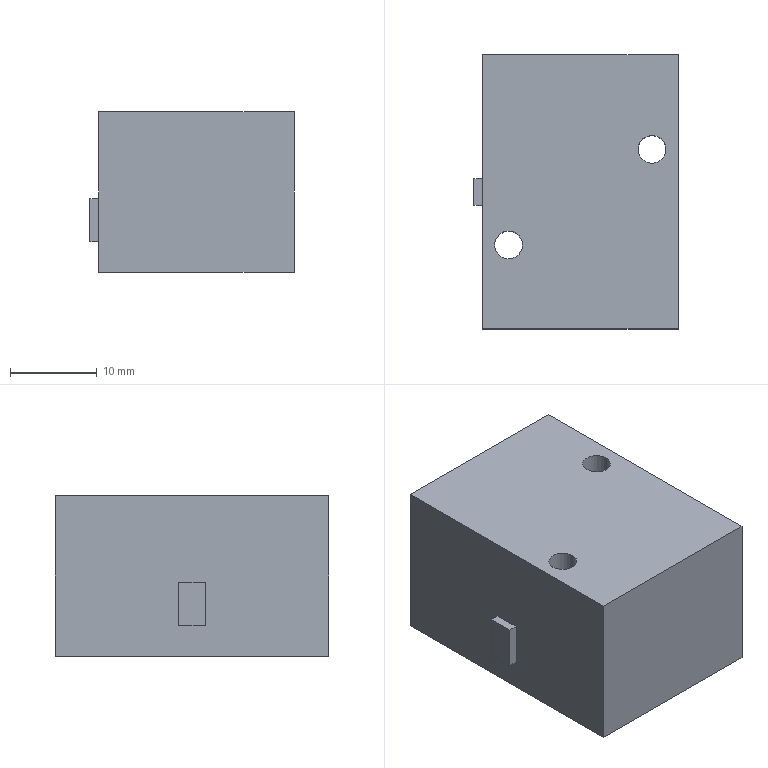Component | SolidWorks | CLS-MechanismAuxiliarySwitch-1 | 1 solid | 15 faces | box 23.5 x 31.5 x 18.5 mm | volume 12829 mm3 | plane 11 | cylinder 4 | commonest cylinder face diameters 3.2 x4 | material 2.0 Galvanized Sheet Q235A
build123d program:
from build123d import *

# Parameters (mm, degrees)
SKETCH1_W            = 22.5
SKETCH1_H            = 31.5
BOSS_EXTRUDE1_DEPTH  = 18.5
SKETCH2_R            = 1.6
CUT_EXTRUDE1_DEPTH   = 27.775
LPATTERN1_COUNT      = 2
LPATTERN1_PITCH      = 16.5
LPATTERN1_COUNT_DIR2 = 2
LPATTERN1_PITCH_DIR2 = 11
SKETCH3_W            = 5
SKETCH3_H            = 3
BOSS_EXTRUDE2_DEPTH  = 1


with BuildPart() as part:
    # Sketch1 → Boss-Extrude1 (new body)
    with BuildSketch(Plane.XY):
        Rectangle(SKETCH1_W, SKETCH1_H)
    extrude(amount=BOSS_EXTRUDE1_DEPTH)

    # Sketch2 → Cut-Extrude1 (cut, through all)
    with BuildSketch(Plane(origin=(0, 0, 0), x_dir=(-1, 0, 0), z_dir=(0, 0, -1))):
        with Locations((-8.25, 4.891)):
            Circle(SKETCH2_R)
    cut_extrude1 = extrude(amount=-CUT_EXTRUDE1_DEPTH, mode=Mode.SUBTRACT)

    # LPattern1: Cut-Extrude1 2 × 2, 2 skipped
    with Locations(*[(-i * LPATTERN1_PITCH, -j * LPATTERN1_PITCH_DIR2, 0) for i in range(LPATTERN1_COUNT) for j in range(LPATTERN1_COUNT_DIR2) if (i, j) not in ((0, 0), (0, 1), (1, 0))]):
        add(cut_extrude1, mode=Mode.SUBTRACT)

    # Sketch3 → Boss-Extrude2 (add)
    with BuildSketch(Plane.ZY.offset(11.25)):
        with Locations((6, 0)):
            Rectangle(SKETCH3_W, SKETCH3_H)
    extrude(amount=BOSS_EXTRUDE2_DEPTH)


solid = part.part

# Placed as in the assembly
solid = solid.moved(Location((19.224, 11.301, -21.501), (0, 0, 0)))
STEP:
#1=COLOUR_RGB('',0.7922,0.8196,0.9333);
#2=FILL_AREA_STYLE_COLOUR('',#1);
#3=FILL_AREA_STYLE('',(#2));
#4=SURFACE_STYLE_FILL_AREA(#3);
#5=SURFACE_SIDE_STYLE('',(#4));
#6=SURFACE_STYLE_USAGE(.BOTH.,#5);
#7=PRESENTATION_STYLE_ASSIGNMENT((#6));
#8=CARTESIAN_POINT('',(0.495,0.2044,-0.1181));
#9=VERTEX_POINT('',#8);
#10=CARTESIAN_POINT('',(0.369,0.2044,-0.1181));
#11=VERTEX_POINT('',#10);
#12=CARTESIAN_POINT('',(0.432,0.2044,-0.1181));
#13=DIRECTION('',(0.,0.,-1.));
#14=DIRECTION('',(-1.,0.,0.));
#15=AXIS2_PLACEMENT_3D('',#12,#13,#14);
#16=CIRCLE('',#15,0.06299);
#17=EDGE_CURVE('',#9,#11,#16,.T.);
#18=ORIENTED_EDGE('',*,*,#17,.F.);
#19=CARTESIAN_POINT('',(0.495,0.2044,-0.8465));
#20=VERTEX_POINT('',#19);
#21=CARTESIAN_POINT('',(0.495,0.2044,-0.1181));
#22=DIRECTION('',(0.,0.,-1.));
#23=VECTOR('',#22,39.37);
#24=LINE('',#21,#23);
#25=EDGE_CURVE('',#9,#20,#24,.T.);
#26=ORIENTED_EDGE('',*,*,#25,.T.);
#27=CARTESIAN_POINT('',(0.369,0.2044,-0.8465));
#28=VERTEX_POINT('',#27);
#29=CARTESIAN_POINT('',(0.432,0.2044,-0.8465));
#30=DIRECTION('',(0.,0.,-1.));
#31=DIRECTION('',(-1.,0.,0.));
#32=AXIS2_PLACEMENT_3D('',#29,#30,#31);
#33=CIRCLE('',#32,0.06299);
#34=EDGE_CURVE('',#20,#28,#33,.T.);
#35=ORIENTED_EDGE('',*,*,#34,.T.);
#36=CARTESIAN_POINT('',(0.369,0.2044,-0.1181));
#37=DIRECTION('',(0.,0.,-1.));
#38=VECTOR('',#37,39.37);
#39=LINE('',#36,#38);
#40=EDGE_CURVE('',#11,#28,#39,.T.);
#41=ORIENTED_EDGE('',*,*,#40,.F.);
#42=EDGE_LOOP('',(#18,#26,#35,#41));
#43=FACE_OUTER_BOUND('',#42,.T.);
#44=CARTESIAN_POINT('',(0.432,0.2044,-0.1181));
#45=DIRECTION('',(0.,0.,-1.));
#46=DIRECTION('',(-1.,0.,0.));
#47=AXIS2_PLACEMENT_3D('',#44,#45,#46);
#48=CYLINDRICAL_SURFACE('',#47,0.06299);
#49=ADVANCED_FACE('',(#43),#48,.F.);
#50=CARTESIAN_POINT('',(1.145,0.6375,-0.1181));
#51=VERTEX_POINT('',#50);
#52=CARTESIAN_POINT('',(1.019,0.6375,-0.1181));
#53=VERTEX_POINT('',#52);
#54=CARTESIAN_POINT('',(1.082,0.6375,-0.1181));
#55=DIRECTION('',(0.,0.,-1.));
#56=DIRECTION('',(-1.,0.,0.));
#57=AXIS2_PLACEMENT_3D('',#54,#55,#56);
#58=CIRCLE('',#57,0.06299);
#59=EDGE_CURVE('',#51,#53,#58,.T.);
#60=ORIENTED_EDGE('',*,*,#59,.F.);
#61=CARTESIAN_POINT('',(1.145,0.6375,-0.8465));
#62=VERTEX_POINT('',#61);
#63=CARTESIAN_POINT('',(1.145,0.6375,-0.1181));
#64=DIRECTION('',(0.,0.,-1.));
#65=VECTOR('',#64,39.37);
#66=LINE('',#63,#65);
#67=EDGE_CURVE('',#51,#62,#66,.T.);
#68=ORIENTED_EDGE('',*,*,#67,.T.);
#69=CARTESIAN_POINT('',(1.019,0.6375,-0.8465));
#70=VERTEX_POINT('',#69);
#71=CARTESIAN_POINT('',(1.082,0.6375,-0.8465));
#72=DIRECTION('',(0.,0.,-1.));
#73=DIRECTION('',(-1.,0.,0.));
#74=AXIS2_PLACEMENT_3D('',#71,#72,#73);
#75=CIRCLE('',#74,0.06299);
#76=EDGE_CURVE('',#62,#70,#75,.T.);
#77=ORIENTED_EDGE('',*,*,#76,.T.);
#78=CARTESIAN_POINT('',(1.019,0.6375,-0.1181));
#79=DIRECTION('',(0.,0.,-1.));
#80=VECTOR('',#79,39.37);
#81=LINE('',#78,#80);
#82=EDGE_CURVE('',#53,#70,#81,.T.);
#83=ORIENTED_EDGE('',*,*,#82,.F.);
#84=EDGE_LOOP('',(#60,#68,#77,#83));
#85=FACE_OUTER_BOUND('',#84,.T.);
#86=CARTESIAN_POINT('',(1.082,0.6375,-0.1181));
#87=DIRECTION('',(0.,0.,-1.));
#88=DIRECTION('',(-1.,0.,0.));
#89=AXIS2_PLACEMENT_3D('',#86,#87,#88);
#90=CYLINDRICAL_SURFACE('',#89,0.06299);
#91=ADVANCED_FACE('',(#85),#90,.F.);
#92=CARTESIAN_POINT('',(0.3139,1.065,-0.8465));
#93=VERTEX_POINT('',#92);
#94=CARTESIAN_POINT('',(0.3139,-0.1752,-0.8465));
#95=VERTEX_POINT('',#94);
#96=CARTESIAN_POINT('',(0.3139,1.065,-0.8465));
#97=DIRECTION('',(0.,-1.,0.));
#98=VECTOR('',#97,39.37);
#99=LINE('',#96,#98);
#100=EDGE_CURVE('',#93,#95,#99,.T.);
#101=ORIENTED_EDGE('',*,*,#100,.T.);
#102=CARTESIAN_POINT('',(0.3139,-0.1752,-0.1181));
#103=VERTEX_POINT('',#102);
#104=CARTESIAN_POINT('',(0.3139,-0.1752,-0.1181));
#105=DIRECTION('',(0.,0.,-1.));
#106=VECTOR('',#105,39.37);
#107=LINE('',#104,#106);
#108=EDGE_CURVE('',#103,#95,#107,.T.);
#109=ORIENTED_EDGE('',*,*,#108,.F.);
#110=CARTESIAN_POINT('',(0.3139,1.065,-0.1181));
#111=VERTEX_POINT('',#110);
#112=CARTESIAN_POINT('',(0.3139,1.065,-0.1181));
#113=DIRECTION('',(0.,-1.,0.));
#114=VECTOR('',#113,39.37);
#115=LINE('',#112,#114);
#116=EDGE_CURVE('',#111,#103,#115,.T.);
#117=ORIENTED_EDGE('',*,*,#116,.F.);
#118=CARTESIAN_POINT('',(0.3139,1.065,-0.1181));
#119=DIRECTION('',(0.,0.,-1.));
#120=VECTOR('',#119,39.37);
#121=LINE('',#118,#120);
#122=EDGE_CURVE('',#111,#93,#121,.T.);
#123=ORIENTED_EDGE('',*,*,#122,.T.);
#124=EDGE_LOOP('',(#101,#109,#117,#123));
#125=FACE_OUTER_BOUND('',#124,.T.);
#126=CARTESIAN_POINT('',(0.3139,0.3859,-0.5118));
#127=VERTEX_POINT('',#126);
#128=CARTESIAN_POINT('',(0.3139,0.504,-0.5118));
#129=VERTEX_POINT('',#128);
#130=CARTESIAN_POINT('',(0.3139,0.504,-0.5118));
#131=DIRECTION('',(0.,1.,-0.));
#132=VECTOR('',#131,39.37);
#133=LINE('',#130,#132);
#134=EDGE_CURVE('',#127,#129,#133,.T.);
#135=ORIENTED_EDGE('',*,*,#134,.F.);
#136=CARTESIAN_POINT('',(0.3139,0.3859,-0.7087));
#137=VERTEX_POINT('',#136);
#138=CARTESIAN_POINT('',(0.3139,0.3859,-0.7087));
#139=DIRECTION('',(0.,0.,1.));
#140=VECTOR('',#139,39.37);
#141=LINE('',#138,#140);
#142=EDGE_CURVE('',#137,#127,#141,.T.);
#143=ORIENTED_EDGE('',*,*,#142,.F.);
#144=CARTESIAN_POINT('',(0.3139,0.504,-0.7087));
#145=VERTEX_POINT('',#144);
#146=CARTESIAN_POINT('',(0.3139,0.504,-0.7087));
#147=DIRECTION('',(0.,-1.,0.));
#148=VECTOR('',#147,39.37);
#149=LINE('',#146,#148);
#150=EDGE_CURVE('',#145,#137,#149,.T.);
#151=ORIENTED_EDGE('',*,*,#150,.F.);
#152=CARTESIAN_POINT('',(0.3139,0.504,-0.7087));
#153=DIRECTION('',(0.,0.,-1.));
#154=VECTOR('',#153,39.37);
#155=LINE('',#152,#154);
#156=EDGE_CURVE('',#129,#145,#155,.T.);
#157=ORIENTED_EDGE('',*,*,#156,.F.);
#158=EDGE_LOOP('',(#135,#143,#151,#157));
#159=FACE_BOUND('',#158,.T.);
#160=CARTESIAN_POINT('',(0.3139,1.065,-0.1181));
#161=DIRECTION('',(1.,0.,0.));
#162=DIRECTION('',(-0.,1.,0.));
#163=AXIS2_PLACEMENT_3D('',#160,#161,#162);
#164=PLANE('',#163);
#165=ADVANCED_FACE('',(#125,#159),#164,.F.);
#166=CARTESIAN_POINT('',(1.2,-0.1752,-0.8465));
#167=VERTEX_POINT('',#166);
#168=CARTESIAN_POINT('',(1.2,-0.1752,-0.8465));
#169=DIRECTION('',(1.,0.,0.));
#170=VECTOR('',#169,39.37);
#171=LINE('',#168,#170);
#172=EDGE_CURVE('',#95,#167,#171,.T.);
#173=ORIENTED_EDGE('',*,*,#172,.T.);
#174=CARTESIAN_POINT('',(1.2,-0.1752,-0.1181));
#175=VERTEX_POINT('',#174);
#176=CARTESIAN_POINT('',(1.2,-0.1752,-0.1181));
#177=DIRECTION('',(0.,0.,-1.));
#178=VECTOR('',#177,39.37);
#179=LINE('',#176,#178);
#180=EDGE_CURVE('',#175,#167,#179,.T.);
#181=ORIENTED_EDGE('',*,*,#180,.F.);
#182=CARTESIAN_POINT('',(1.2,-0.1752,-0.1181));
#183=DIRECTION('',(1.,0.,0.));
#184=VECTOR('',#183,39.37);
#185=LINE('',#182,#184);
#186=EDGE_CURVE('',#103,#175,#185,.T.);
#187=ORIENTED_EDGE('',*,*,#186,.F.);
#188=ORIENTED_EDGE('',*,*,#108,.T.);
#189=EDGE_LOOP('',(#173,#181,#187,#188));
#190=FACE_OUTER_BOUND('',#189,.T.);
#191=CARTESIAN_POINT('',(1.2,-0.1752,-0.1181));
#192=DIRECTION('',(0.,1.,0.));
#193=DIRECTION('',(0.,0.,1.));
#194=AXIS2_PLACEMENT_3D('',#191,#192,#193);
#195=PLANE('',#194);
#196=ADVANCED_FACE('',(#190),#195,.F.);
#197=CARTESIAN_POINT('',(1.2,1.065,-0.8465));
#198=VERTEX_POINT('',#197);
#199=CARTESIAN_POINT('',(1.2,1.065,-0.8465));
#200=DIRECTION('',(-0.,1.,0.));
#201=VECTOR('',#200,39.37);
#202=LINE('',#199,#201);
#203=EDGE_CURVE('',#167,#198,#202,.T.);
#204=ORIENTED_EDGE('',*,*,#203,.T.);
#205=CARTESIAN_POINT('',(1.2,1.065,-0.1181));
#206=VERTEX_POINT('',#205);
#207=CARTESIAN_POINT('',(1.2,1.065,-0.1181));
#208=DIRECTION('',(0.,0.,-1.));
#209=VECTOR('',#208,39.37);
#210=LINE('',#207,#209);
#211=EDGE_CURVE('',#206,#198,#210,.T.);
#212=ORIENTED_EDGE('',*,*,#211,.F.);
#213=CARTESIAN_POINT('',(1.2,1.065,-0.1181));
#214=DIRECTION('',(-0.,1.,0.));
#215=VECTOR('',#214,39.37);
#216=LINE('',#213,#215);
#217=EDGE_CURVE('',#175,#206,#216,.T.);
#218=ORIENTED_EDGE('',*,*,#217,.F.);
#219=ORIENTED_EDGE('',*,*,#180,.T.);
#220=EDGE_LOOP('',(#204,#212,#218,#219));
#221=FACE_OUTER_BOUND('',#220,.T.);
#222=CARTESIAN_POINT('',(1.2,1.065,-0.1181));
#223=DIRECTION('',(-1.,-0.,0.));
#224=DIRECTION('',(0.,-1.,0.));
#225=AXIS2_PLACEMENT_3D('',#222,#223,#224);
#226=PLANE('',#225);
#227=ADVANCED_FACE('',(#221),#226,.F.);
#228=CARTESIAN_POINT('',(1.2,1.065,-0.8465));
#229=DIRECTION('',(-1.,-0.,0.));
#230=VECTOR('',#229,39.37);
#231=LINE('',#228,#230);
#232=EDGE_CURVE('',#198,#93,#231,.T.);
#233=ORIENTED_EDGE('',*,*,#232,.T.);
#234=ORIENTED_EDGE('',*,*,#122,.F.);
#235=CARTESIAN_POINT('',(1.2,1.065,-0.1181));
#236=DIRECTION('',(-1.,-0.,0.));
#237=VECTOR('',#236,39.37);
#238=LINE('',#235,#237);
#239=EDGE_CURVE('',#206,#111,#238,.T.);
#240=ORIENTED_EDGE('',*,*,#239,.F.);
#241=ORIENTED_EDGE('',*,*,#211,.T.);
#242=EDGE_LOOP('',(#233,#234,#240,#241));
#243=FACE_OUTER_BOUND('',#242,.T.);
#244=CARTESIAN_POINT('',(1.2,1.065,-0.1181));
#245=DIRECTION('',(0.,-1.,0.));
#246=DIRECTION('',(1.,0.,0.));
#247=AXIS2_PLACEMENT_3D('',#244,#245,#246);
#248=PLANE('',#247);
#249=ADVANCED_FACE('',(#243),#248,.F.);
#250=CARTESIAN_POINT('',(0.432,0.2044,-0.1181));
#251=DIRECTION('',(0.,0.,-1.));
#252=DIRECTION('',(-1.,0.,0.));
#253=AXIS2_PLACEMENT_3D('',#250,#251,#252);
#254=CIRCLE('',#253,0.06299);
#255=EDGE_CURVE('',#11,#9,#254,.T.);
#256=ORIENTED_EDGE('',*,*,#255,.T.);
#257=ORIENTED_EDGE('',*,*,#17,.T.);
#258=EDGE_LOOP('',(#256,#257));
#259=FACE_BOUND('',#258,.T.);
#260=CARTESIAN_POINT('',(1.082,0.6375,-0.1181));
#261=DIRECTION('',(0.,0.,-1.));
#262=DIRECTION('',(-1.,0.,0.));
#263=AXIS2_PLACEMENT_3D('',#260,#261,#262);
#264=CIRCLE('',#263,0.06299);
#265=EDGE_CURVE('',#53,#51,#264,.T.);
#266=ORIENTED_EDGE('',*,*,#265,.T.);
#267=ORIENTED_EDGE('',*,*,#59,.T.);
#268=EDGE_LOOP('',(#266,#267));
#269=FACE_BOUND('',#268,.T.);
#270=ORIENTED_EDGE('',*,*,#116,.T.);
#271=ORIENTED_EDGE('',*,*,#186,.T.);
#272=ORIENTED_EDGE('',*,*,#217,.T.);
#273=ORIENTED_EDGE('',*,*,#239,.T.);
#274=EDGE_LOOP('',(#270,#271,#272,#273));
#275=FACE_OUTER_BOUND('',#274,.T.);
#276=CARTESIAN_POINT('',(0.3139,-0.1752,-0.1181));
#277=DIRECTION('',(0.,0.,-1.));
#278=DIRECTION('',(-1.,0.,0.));
#279=AXIS2_PLACEMENT_3D('',#276,#277,#278);
#280=PLANE('',#279);
#281=ADVANCED_FACE('',(#259,#269,#275),#280,.F.);
#282=CARTESIAN_POINT('',(0.432,0.2044,-0.8465));
#283=DIRECTION('',(0.,0.,-1.));
#284=DIRECTION('',(-1.,0.,0.));
#285=AXIS2_PLACEMENT_3D('',#282,#283,#284);
#286=CIRCLE('',#285,0.06299);
#287=EDGE_CURVE('',#28,#20,#286,.T.);
#288=ORIENTED_EDGE('',*,*,#287,.F.);
#289=ORIENTED_EDGE('',*,*,#34,.F.);
#290=EDGE_LOOP('',(#288,#289));
#291=FACE_BOUND('',#290,.T.);
#292=CARTESIAN_POINT('',(1.082,0.6375,-0.8465));
#293=DIRECTION('',(0.,0.,-1.));
#294=DIRECTION('',(-1.,0.,0.));
#295=AXIS2_PLACEMENT_3D('',#292,#293,#294);
#296=CIRCLE('',#295,0.06299);
#297=EDGE_CURVE('',#70,#62,#296,.T.);
#298=ORIENTED_EDGE('',*,*,#297,.F.);
#299=ORIENTED_EDGE('',*,*,#76,.F.);
#300=EDGE_LOOP('',(#298,#299));
#301=FACE_BOUND('',#300,.T.);
#302=ORIENTED_EDGE('',*,*,#100,.F.);
#303=ORIENTED_EDGE('',*,*,#232,.F.);
#304=ORIENTED_EDGE('',*,*,#203,.F.);
#305=ORIENTED_EDGE('',*,*,#172,.F.);
#306=EDGE_LOOP('',(#302,#303,#304,#305));
#307=FACE_OUTER_BOUND('',#306,.T.);
#308=CARTESIAN_POINT('',(0.3139,-0.1752,-0.8465));
#309=DIRECTION('',(0.,0.,-1.));
#310=DIRECTION('',(-1.,0.,0.));
#311=AXIS2_PLACEMENT_3D('',#308,#309,#310);
#312=PLANE('',#311);
#313=ADVANCED_FACE('',(#291,#301,#307),#312,.T.);
#314=ORIENTED_EDGE('',*,*,#67,.F.);
#315=ORIENTED_EDGE('',*,*,#265,.F.);
#316=ORIENTED_EDGE('',*,*,#82,.T.);
#317=ORIENTED_EDGE('',*,*,#297,.T.);
#318=EDGE_LOOP('',(#314,#315,#316,#317));
#319=FACE_OUTER_BOUND('',#318,.T.);
#320=CARTESIAN_POINT('',(1.082,0.6375,-0.1181));
#321=DIRECTION('',(0.,0.,-1.));
#322=DIRECTION('',(-1.,0.,0.));
#323=AXIS2_PLACEMENT_3D('',#320,#321,#322);
#324=CYLINDRICAL_SURFACE('',#323,0.06299);
#325=ADVANCED_FACE('',(#319),#324,.F.);
#326=ORIENTED_EDGE('',*,*,#25,.F.);
#327=ORIENTED_EDGE('',*,*,#255,.F.);
#328=ORIENTED_EDGE('',*,*,#40,.T.);
#329=ORIENTED_EDGE('',*,*,#287,.T.);
#330=EDGE_LOOP('',(#326,#327,#328,#329));
#331=FACE_OUTER_BOUND('',#330,.T.);
#332=CARTESIAN_POINT('',(0.432,0.2044,-0.1181));
#333=DIRECTION('',(0.,0.,-1.));
#334=DIRECTION('',(-1.,0.,0.));
#335=AXIS2_PLACEMENT_3D('',#332,#333,#334);
#336=CYLINDRICAL_SURFACE('',#335,0.06299);
#337=ADVANCED_FACE('',(#331),#336,.F.);
#338=ORIENTED_EDGE('',*,*,#134,.T.);
#339=CARTESIAN_POINT('',(0.2746,0.504,-0.5118));
#340=VERTEX_POINT('',#339);
#341=CARTESIAN_POINT('',(0.2746,0.504,-0.5118));
#342=DIRECTION('',(1.,0.,0.));
#343=VECTOR('',#342,39.37);
#344=LINE('',#341,#343);
#345=EDGE_CURVE('',#340,#129,#344,.T.);
#346=ORIENTED_EDGE('',*,*,#345,.F.);
#347=CARTESIAN_POINT('',(0.2746,0.3859,-0.5118));
#348=VERTEX_POINT('',#347);
#349=CARTESIAN_POINT('',(0.2746,0.504,-0.5118));
#350=DIRECTION('',(0.,1.,-0.));
#351=VECTOR('',#350,39.37);
#352=LINE('',#349,#351);
#353=EDGE_CURVE('',#348,#340,#352,.T.);
#354=ORIENTED_EDGE('',*,*,#353,.F.);
#355=CARTESIAN_POINT('',(0.2746,0.3859,-0.5118));
#356=DIRECTION('',(1.,0.,0.));
#357=VECTOR('',#356,39.37);
#358=LINE('',#355,#357);
#359=EDGE_CURVE('',#348,#127,#358,.T.);
#360=ORIENTED_EDGE('',*,*,#359,.T.);
#361=EDGE_LOOP('',(#338,#346,#354,#360));
#362=FACE_OUTER_BOUND('',#361,.T.);
#363=CARTESIAN_POINT('',(0.2746,0.504,-0.5118));
#364=DIRECTION('',(0.,-0.,-1.));
#365=DIRECTION('',(0.,1.,-0.));
#366=AXIS2_PLACEMENT_3D('',#363,#364,#365);
#367=PLANE('',#366);
#368=ADVANCED_FACE('',(#362),#367,.F.);
#369=ORIENTED_EDGE('',*,*,#156,.T.);
#370=CARTESIAN_POINT('',(0.2746,0.504,-0.7087));
#371=VERTEX_POINT('',#370);
#372=CARTESIAN_POINT('',(0.2746,0.504,-0.7087));
#373=DIRECTION('',(1.,0.,0.));
#374=VECTOR('',#373,39.37);
#375=LINE('',#372,#374);
#376=EDGE_CURVE('',#371,#145,#375,.T.);
#377=ORIENTED_EDGE('',*,*,#376,.F.);
#378=CARTESIAN_POINT('',(0.2746,0.504,-0.7087));
#379=DIRECTION('',(0.,0.,-1.));
#380=VECTOR('',#379,39.37);
#381=LINE('',#378,#380);
#382=EDGE_CURVE('',#340,#371,#381,.T.);
#383=ORIENTED_EDGE('',*,*,#382,.F.);
#384=ORIENTED_EDGE('',*,*,#345,.T.);
#385=EDGE_LOOP('',(#369,#377,#383,#384));
#386=FACE_OUTER_BOUND('',#385,.T.);
#387=CARTESIAN_POINT('',(0.2746,0.504,-0.7087));
#388=DIRECTION('',(0.,-1.,0.));
#389=DIRECTION('',(1.,0.,0.));
#390=AXIS2_PLACEMENT_3D('',#387,#388,#389);
#391=PLANE('',#390);
#392=ADVANCED_FACE('',(#386),#391,.F.);
#393=ORIENTED_EDGE('',*,*,#150,.T.);
#394=CARTESIAN_POINT('',(0.2746,0.3859,-0.7087));
#395=VERTEX_POINT('',#394);
#396=CARTESIAN_POINT('',(0.2746,0.3859,-0.7087));
#397=DIRECTION('',(1.,0.,0.));
#398=VECTOR('',#397,39.37);
#399=LINE('',#396,#398);
#400=EDGE_CURVE('',#395,#137,#399,.T.);
#401=ORIENTED_EDGE('',*,*,#400,.F.);
#402=CARTESIAN_POINT('',(0.2746,0.504,-0.7087));
#403=DIRECTION('',(0.,-1.,0.));
#404=VECTOR('',#403,39.37);
#405=LINE('',#402,#404);
#406=EDGE_CURVE('',#371,#395,#405,.T.);
#407=ORIENTED_EDGE('',*,*,#406,.F.);
#408=ORIENTED_EDGE('',*,*,#376,.T.);
#409=EDGE_LOOP('',(#393,#401,#407,#408));
#410=FACE_OUTER_BOUND('',#409,.T.);
#411=CARTESIAN_POINT('',(0.2746,0.504,-0.7087));
#412=DIRECTION('',(-0.,0.,1.));
#413=DIRECTION('',(0.,-1.,0.));
#414=AXIS2_PLACEMENT_3D('',#411,#412,#413);
#415=PLANE('',#414);
#416=ADVANCED_FACE('',(#410),#415,.F.);
#417=ORIENTED_EDGE('',*,*,#142,.T.);
#418=ORIENTED_EDGE('',*,*,#359,.F.);
#419=CARTESIAN_POINT('',(0.2746,0.3859,-0.7087));
#420=DIRECTION('',(0.,0.,1.));
#421=VECTOR('',#420,39.37);
#422=LINE('',#419,#421);
#423=EDGE_CURVE('',#395,#348,#422,.T.);
#424=ORIENTED_EDGE('',*,*,#423,.F.);
#425=ORIENTED_EDGE('',*,*,#400,.T.);
#426=EDGE_LOOP('',(#417,#418,#424,#425));
#427=FACE_OUTER_BOUND('',#426,.T.);
#428=CARTESIAN_POINT('',(0.2746,0.3859,-0.7087));
#429=DIRECTION('',(-0.,1.,0.));
#430=DIRECTION('',(-1.,-0.,0.));
#431=AXIS2_PLACEMENT_3D('',#428,#429,#430);
#432=PLANE('',#431);
#433=ADVANCED_FACE('',(#427),#432,.F.);
#434=ORIENTED_EDGE('',*,*,#353,.T.);
#435=ORIENTED_EDGE('',*,*,#382,.T.);
#436=ORIENTED_EDGE('',*,*,#406,.T.);
#437=ORIENTED_EDGE('',*,*,#423,.T.);
#438=EDGE_LOOP('',(#434,#435,#436,#437));
#439=FACE_OUTER_BOUND('',#438,.T.);
#440=CARTESIAN_POINT('',(0.2746,0.3859,-0.5118));
#441=DIRECTION('',(-1.,0.,0.));
#442=DIRECTION('',(0.,0.,1.));
#443=AXIS2_PLACEMENT_3D('',#440,#441,#442);
#444=PLANE('',#443);
#445=ADVANCED_FACE('',(#439),#444,.T.);
#446=CLOSED_SHELL('',(#49,#91,#165,#196,#227,#249,#281,#313,#325,#337,#368,#392,#416,#433,#445));
#447=MANIFOLD_SOLID_BREP('',#446);
#448=STYLED_ITEM('',(#7),#447);
#449=PRESENTATION_LAYER_ASSIGNMENT('','',(#448));
#450=CARTESIAN_POINT('',(0.,0.,0.));
#451=DIRECTION('',(0.,0.,1.));
#452=DIRECTION('',(1.,0.,0.));
#453=AXIS2_PLACEMENT_3D('',#450,#451,#452);
#454=(LENGTH_UNIT()NAMED_UNIT(*)SI_UNIT($,.METRE.));
#455=LENGTH_MEASURE_WITH_UNIT(LENGTH_MEASURE(0.0254),#454);
#456=DIMENSIONAL_EXPONENTS(1.,0.,0.,0.,0.,0.,0.);
#457=(CONVERSION_BASED_UNIT('',#455)LENGTH_UNIT()NAMED_UNIT(#456));
#458=UNCERTAINTY_MEASURE_WITH_UNIT(LENGTH_MEASURE(0.00001),#457,'','');
#459=(NAMED_UNIT(*)PLANE_ANGLE_UNIT()SI_UNIT($,.RADIAN.));
#460=(NAMED_UNIT(*)SI_UNIT($,.STERADIAN.)SOLID_ANGLE_UNIT());
#461=(GEOMETRIC_REPRESENTATION_CONTEXT(3)GLOBAL_UNCERTAINTY_ASSIGNED_CONTEXT((#458))GLOBAL_UNIT_ASSIGNED_CONTEXT((#457,#459,#460))REPRESENTATION_CONTEXT('',''));
#462=ADVANCED_BREP_SHAPE_REPRESENTATION('',(#447,#453),#461);
#463=(LENGTH_UNIT()NAMED_UNIT(*)SI_UNIT($,.METRE.));
#464=LENGTH_MEASURE_WITH_UNIT(LENGTH_MEASURE(0.0254),#463);
#465=DIMENSIONAL_EXPONENTS(1.,0.,0.,0.,0.,0.,0.);
#466=(CONVERSION_BASED_UNIT('',#464)LENGTH_UNIT()NAMED_UNIT(#465));
#467=UNCERTAINTY_MEASURE_WITH_UNIT(LENGTH_MEASURE(0.00001),#466,'','');
#468=(NAMED_UNIT(*)PLANE_ANGLE_UNIT()SI_UNIT($,.RADIAN.));
#469=(NAMED_UNIT(*)SI_UNIT($,.STERADIAN.)SOLID_ANGLE_UNIT());
#470=(GEOMETRIC_REPRESENTATION_CONTEXT(3)GLOBAL_UNCERTAINTY_ASSIGNED_CONTEXT((#467))GLOBAL_UNIT_ASSIGNED_CONTEXT((#466,#468,#469))REPRESENTATION_CONTEXT('',''));
#471=MECHANICAL_DESIGN_GEOMETRIC_PRESENTATION_REPRESENTATION('',(#448),#470);